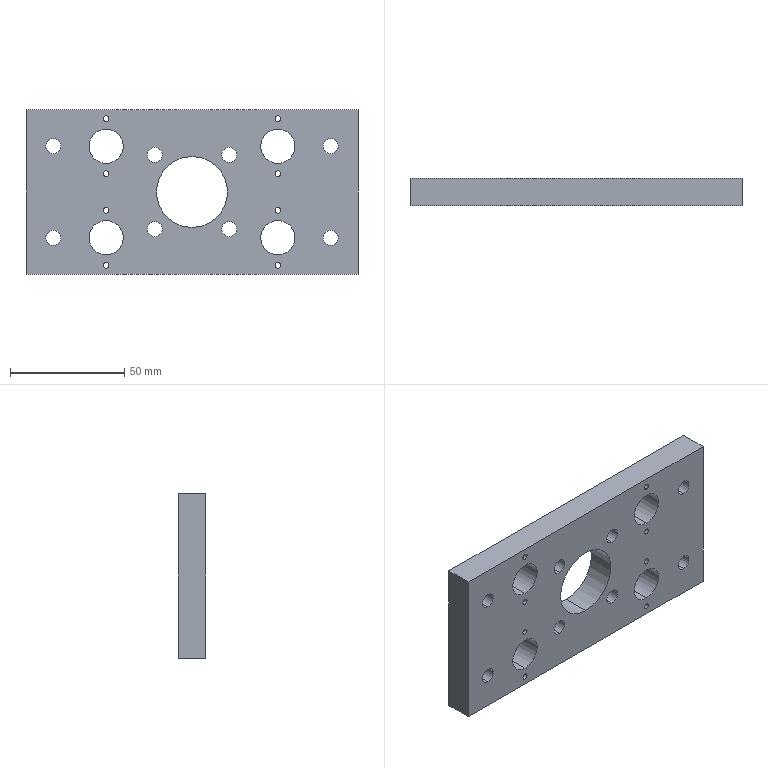Component | SolidWorks | F12529-M5101-1 | 1 solid | 72 faces | box 145 x 12 x 72 mm | volume 101065 mm3 | cylinder 58 | plane 14 | commonest cylinder face diameters 2.5 x16 6.6 x16 11 x16 15 x8 31 x2
build123d program:
from build123d import *

# Parameters (mm, degrees)
SKETCH1_W                                            = 145
SKETCH1_H                                            = 72
EXTRUDE1_DEPTH                                       = 12
SKETCH3_R                                            = 7.5
CUT_EXTRUDE1_DEPTH                                   = 82.831
M6_HEX_SOCKET_HEAD_CAP_SCREW_COUNTERBORE_D           = 6.6
M6_HEX_SOCKET_HEAD_CAP_SCREW_COUNTERBORE_CBORE_D     = 11
M6_HEX_SOCKET_HEAD_CAP_SCREW_COUNTERBORE_CBORE_DEPTH = 6
SKETCH9_R                                            = 15.5
CUT_EXTRUDE2_DEPTH                                   = 82.831
COUNTERBORE_FOR_M6_HEX_SOCKET_HEAD_CAP_S_D           = 6.6
COUNTERBORE_FOR_M6_HEX_SOCKET_HEAD_CAP_S_CBORE_D     = 11
COUNTERBORE_FOR_M6_HEX_SOCKET_HEAD_CAP_S_CBORE_DEPTH = 6
M3_TAPPED_HOLE1_D                                    = 2.5
MIRROR5_COPY_1_D                                     = 2.5


with BuildPart() as part:
    # Sketch1 → Extrude1 (new body)
    with BuildSketch(Plane(origin=(0, 0, 0), x_dir=(1, 0, 0), z_dir=(0, 1, 0))):
        Rectangle(SKETCH1_W, SKETCH1_H)
    extrude(amount=EXTRUDE1_DEPTH)

    # Sketch3 → Cut-Extrude1 (cut, through all)
    with BuildSketch(Plane(origin=(0, 12, 0), x_dir=(1, 0, 0), z_dir=(0, 1, 0))):
        with Locations(Location((37.5, 20, 0), (0, 0, 270))):
            Circle(SKETCH3_R)
        with Locations(Location((37.5, -20, 0), (0, 0, 270))):
            Circle(SKETCH3_R)
    cut_extrude1 = extrude(amount=-CUT_EXTRUDE1_DEPTH, mode=Mode.SUBTRACT)

    # Mirror1: Cut-Extrude1 across plane
    add(cut_extrude1.mirror(Plane(origin=(0, 0, 0), x_dir=(0, 0, 1), z_dir=(1, 0, 0))), mode=Mode.SUBTRACT)

    # M6 Hex Socket Head Cap Screw Counterbore (through all)
    with Locations(Plane(origin=(0, 12, 0), x_dir=(-1, 0, 0), z_dir=(0, 1, 0))):
        with Locations((-16.25, -16.25), (-16.25, 16.25)):
            m6_hex_socket_head_cap_screw_counterbore = CounterBoreHole(M6_HEX_SOCKET_HEAD_CAP_SCREW_COUNTERBORE_D / 2, M6_HEX_SOCKET_HEAD_CAP_SCREW_COUNTERBORE_CBORE_D / 2, M6_HEX_SOCKET_HEAD_CAP_SCREW_COUNTERBORE_CBORE_DEPTH)

    # Mirror2: M6 Hex Socket Head Cap Screw Counterbore across plane
    add(m6_hex_socket_head_cap_screw_counterbore.mirror(Plane(origin=(0, 0, 0), x_dir=(0, 0, 1), z_dir=(1, 0, 0))), mode=Mode.SUBTRACT)

    # Sketch9 → Cut-Extrude2 (cut, through all)
    with BuildSketch(Plane(origin=(0, 12, 0), x_dir=(1, 0, 0), z_dir=(0, 1, 0))):
        with Locations(Location((0, 0, 0), (0, 0, 270))):
            Circle(SKETCH9_R)
    extrude(amount=-CUT_EXTRUDE2_DEPTH, mode=Mode.SUBTRACT)

    # Counterbore for M6 Hex Socket Head Cap S (through all)
    with Locations(Plane(origin=(0, 12, 0), x_dir=(-1, 0, 0), z_dir=(0, 1, 0))):
        with Locations((-60.5, -20), (-60.5, 20)):
            counterbore_for_m6_hex_socket_head_cap_s = CounterBoreHole(COUNTERBORE_FOR_M6_HEX_SOCKET_HEAD_CAP_S_D / 2, COUNTERBORE_FOR_M6_HEX_SOCKET_HEAD_CAP_S_CBORE_D / 2, COUNTERBORE_FOR_M6_HEX_SOCKET_HEAD_CAP_S_CBORE_DEPTH)

    # Mirror3: Counterbore for M6 Hex Socket Head Cap S across plane
    add(counterbore_for_m6_hex_socket_head_cap_s.mirror(Plane(origin=(0, 0, 0), x_dir=(0, 0, 1), z_dir=(1, 0, 0))), mode=Mode.SUBTRACT)

    # M3 Tapped Hole1 (through all)
    with Locations(Plane.XZ):
        with Locations((37.5, 32), (37.5, 8)):
            m3_tapped_hole1 = Hole(M3_TAPPED_HOLE1_D / 2)

    # Mirror4: M3 Tapped Hole1 across plane
    add(m3_tapped_hole1.mirror(Plane.XY), mode=Mode.SUBTRACT)

    # Mirror5: M3 Tapped Hole1 across plane
    add(m3_tapped_hole1.mirror(Plane(origin=(0, 0, 0), x_dir=(0, 0, 1), z_dir=(1, 0, 0))), mode=Mode.SUBTRACT)

    # Mirror5 copy 1 (through all)
    with Locations(Plane(origin=(0, 0, 0), x_dir=(-1, 0, 0), z_dir=(0, -1, 0))):
        with Locations((37.5, 32), (37.5, 8)):
            Hole(MIRROR5_COPY_1_D / 2)


solid = part.part